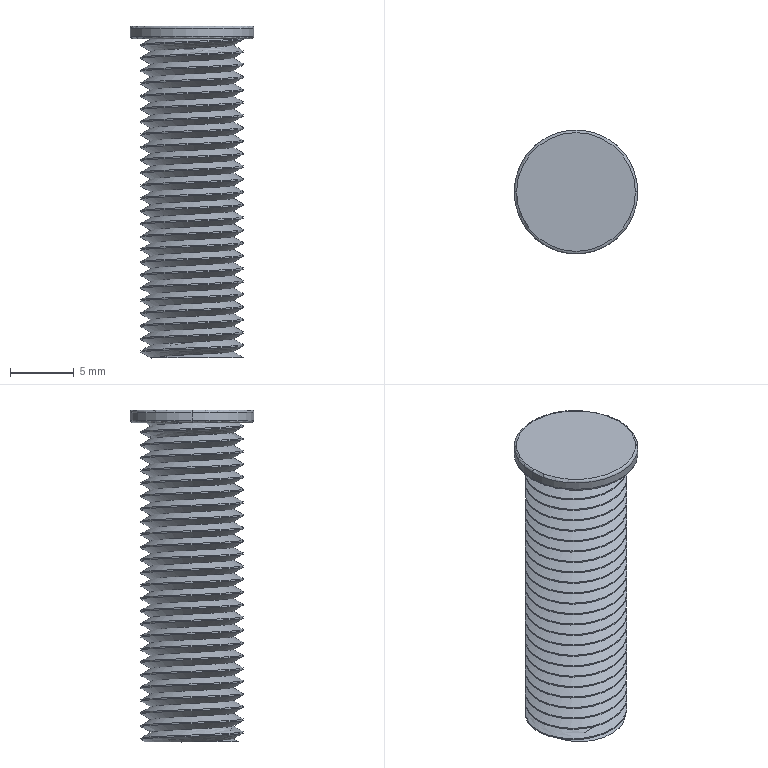Component | SolidWorks | M8X25WeldScrew-1 | 1 solid | 63 faces | volume 1124 mm3 | cylinder 54 | torus 4 | plane 3 | spline 2 | commonest cylinder face diameters 8 x52 9.7 x2